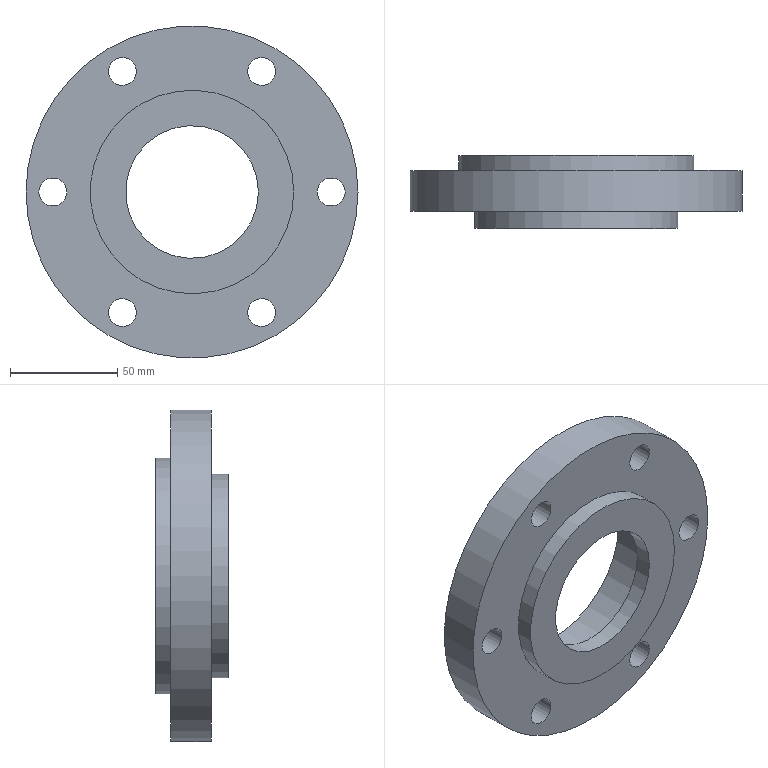Component | NX | END_CAP2 | 1 solid | 18 faces | volume 290876 mm3 | cylinder 12 | plane 6 | commonest cylinder face diameters 13 x6 155 x1 95 x1 110 x1 99 x1 85 x1 62 x1